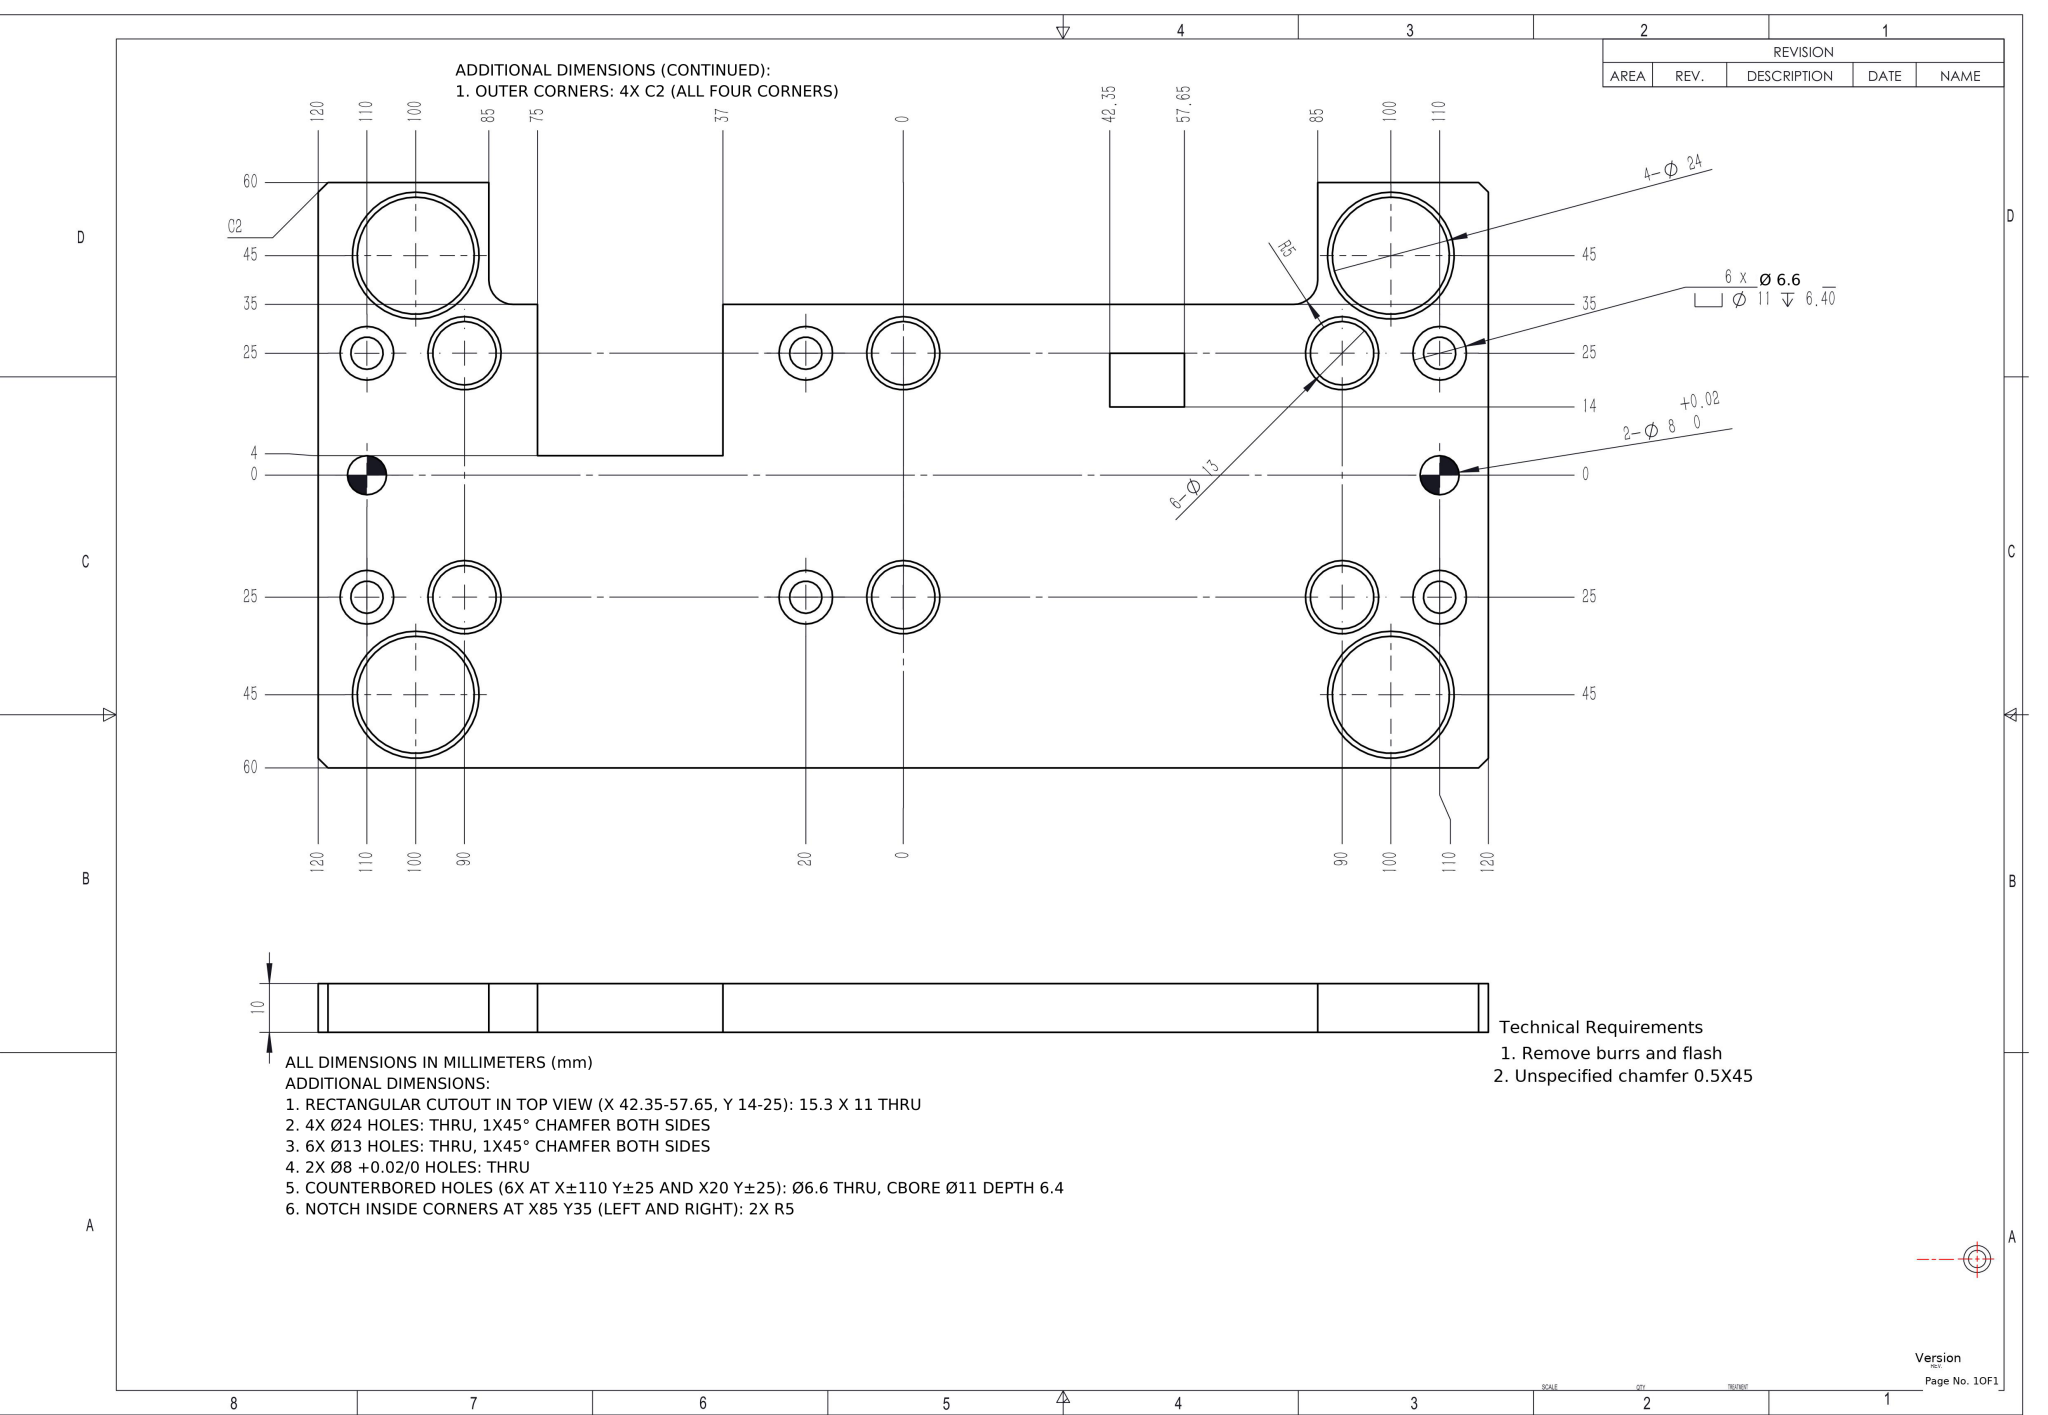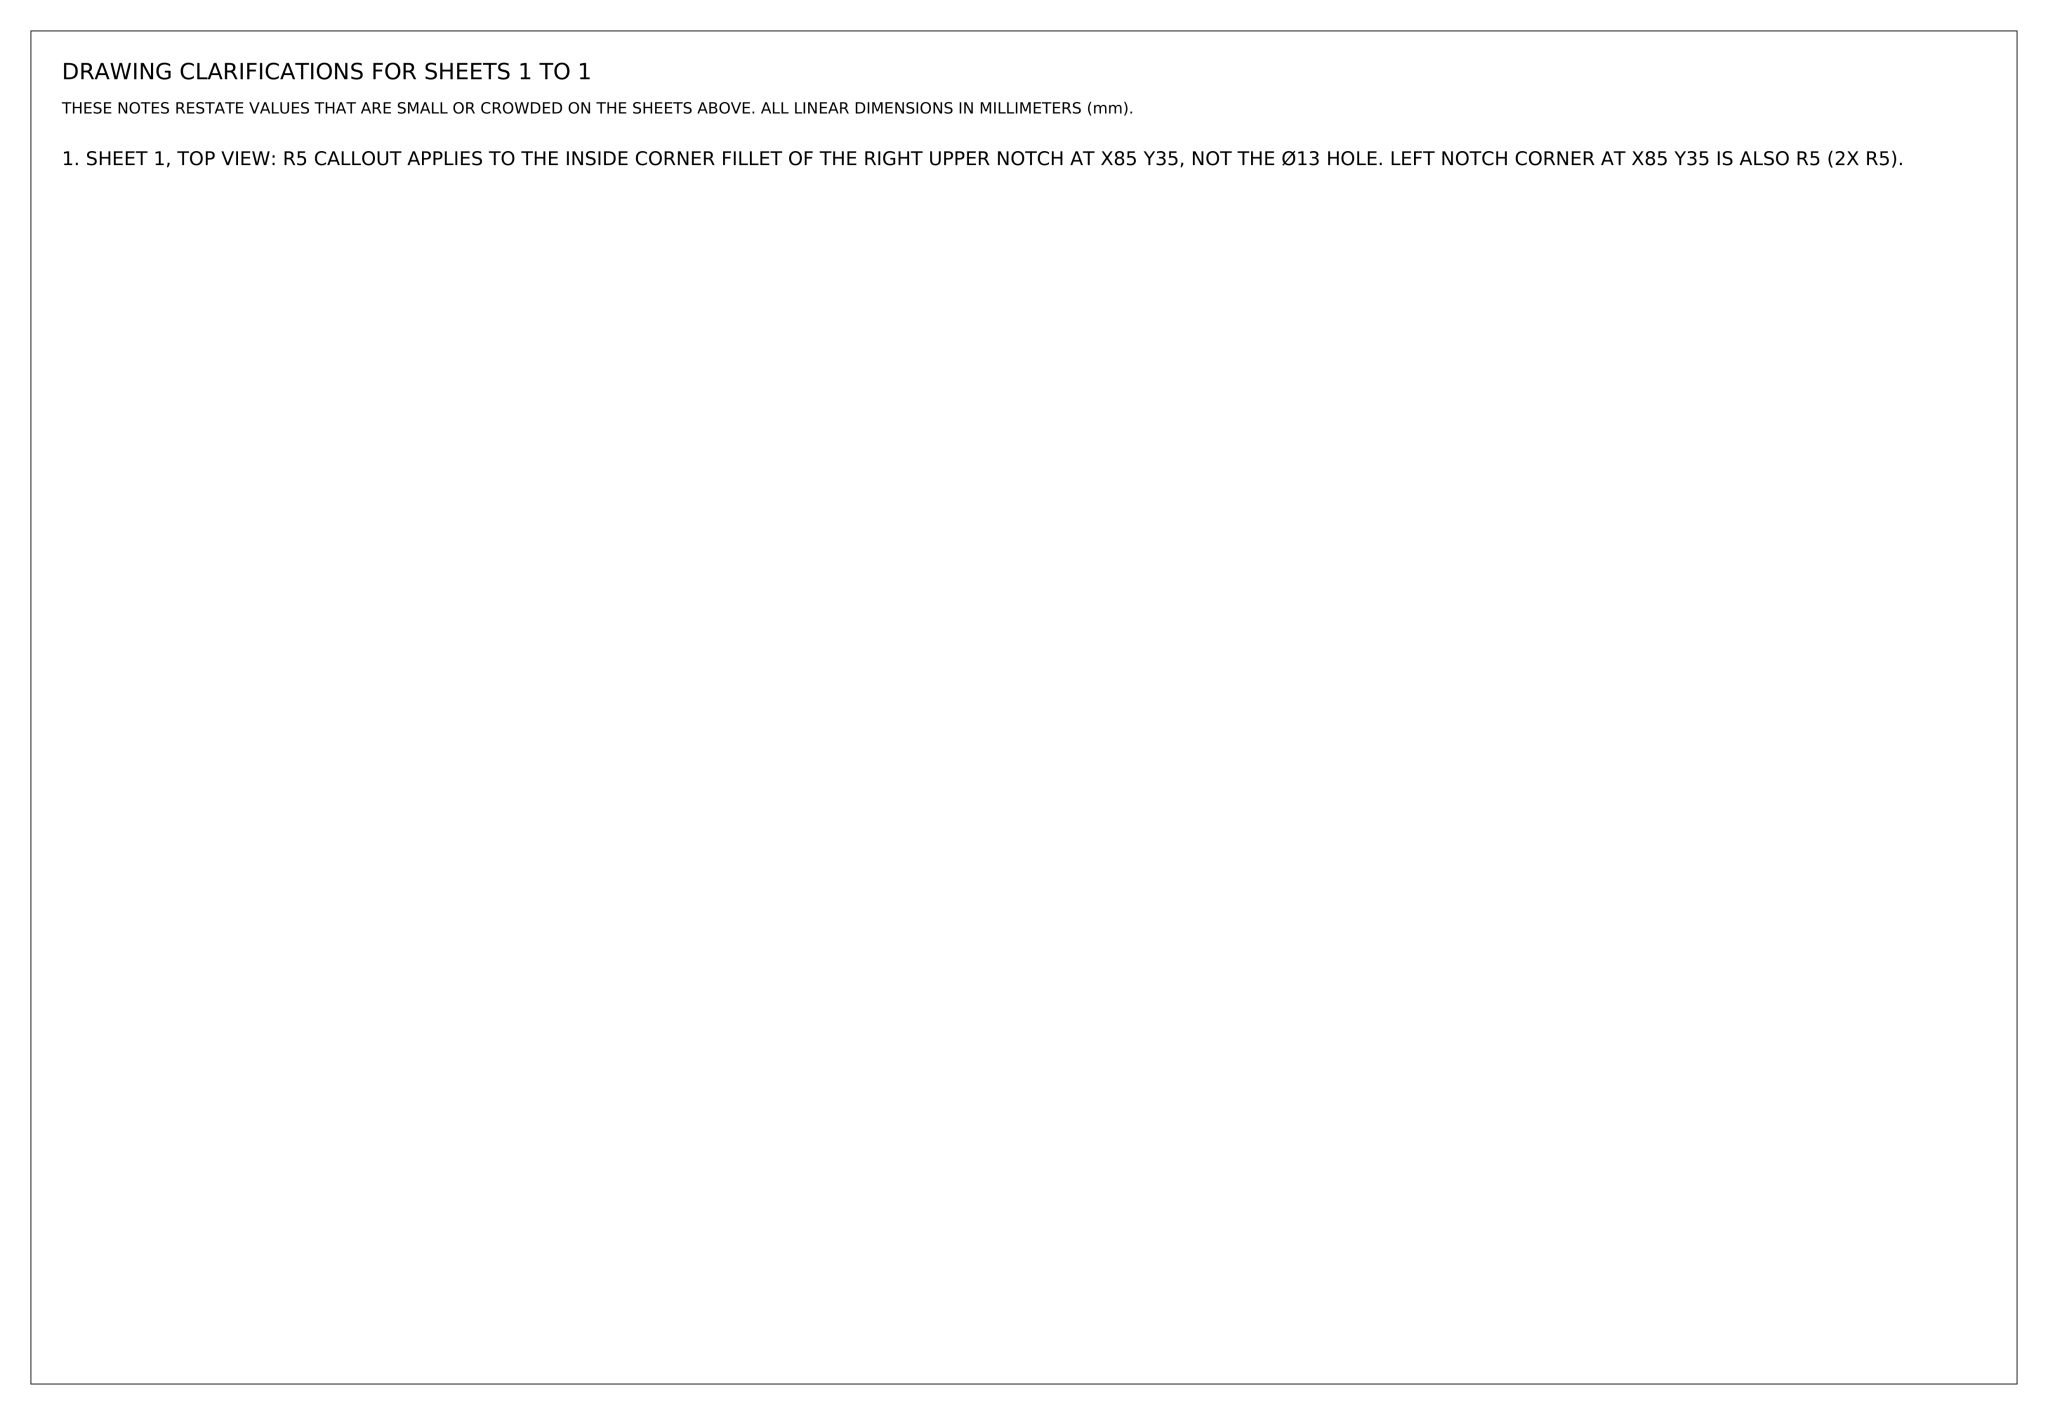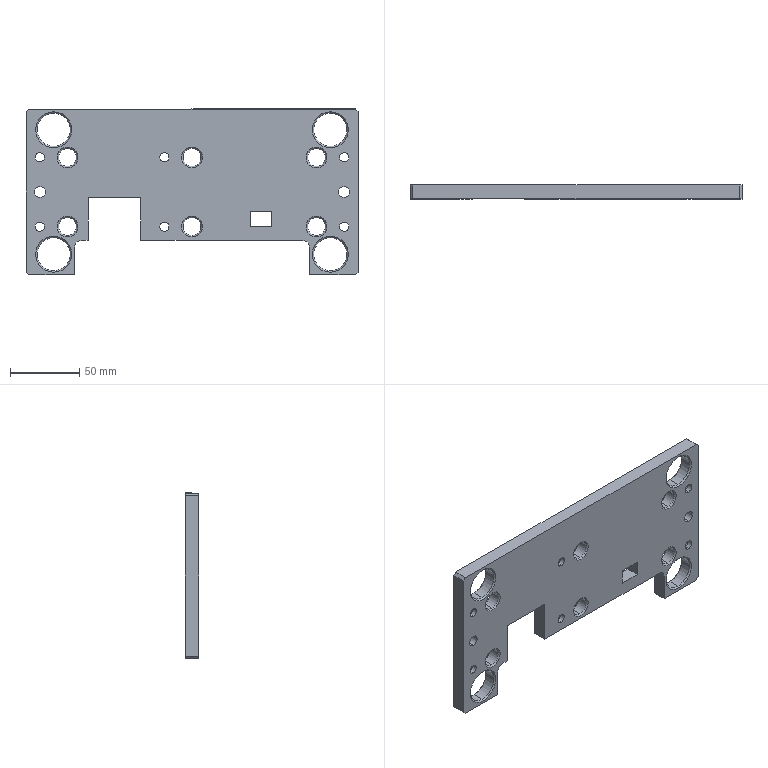Part | NX | mm | 1 solid | 118 faces | box 240 x 10 x 120 mm | volume 200044 mm3 | cylinder 50 | cone 40 | plane 28 | commonest cylinder face diameters 11 x12 6.6 x12 13 x12 24 x8 8 x4 10 x2